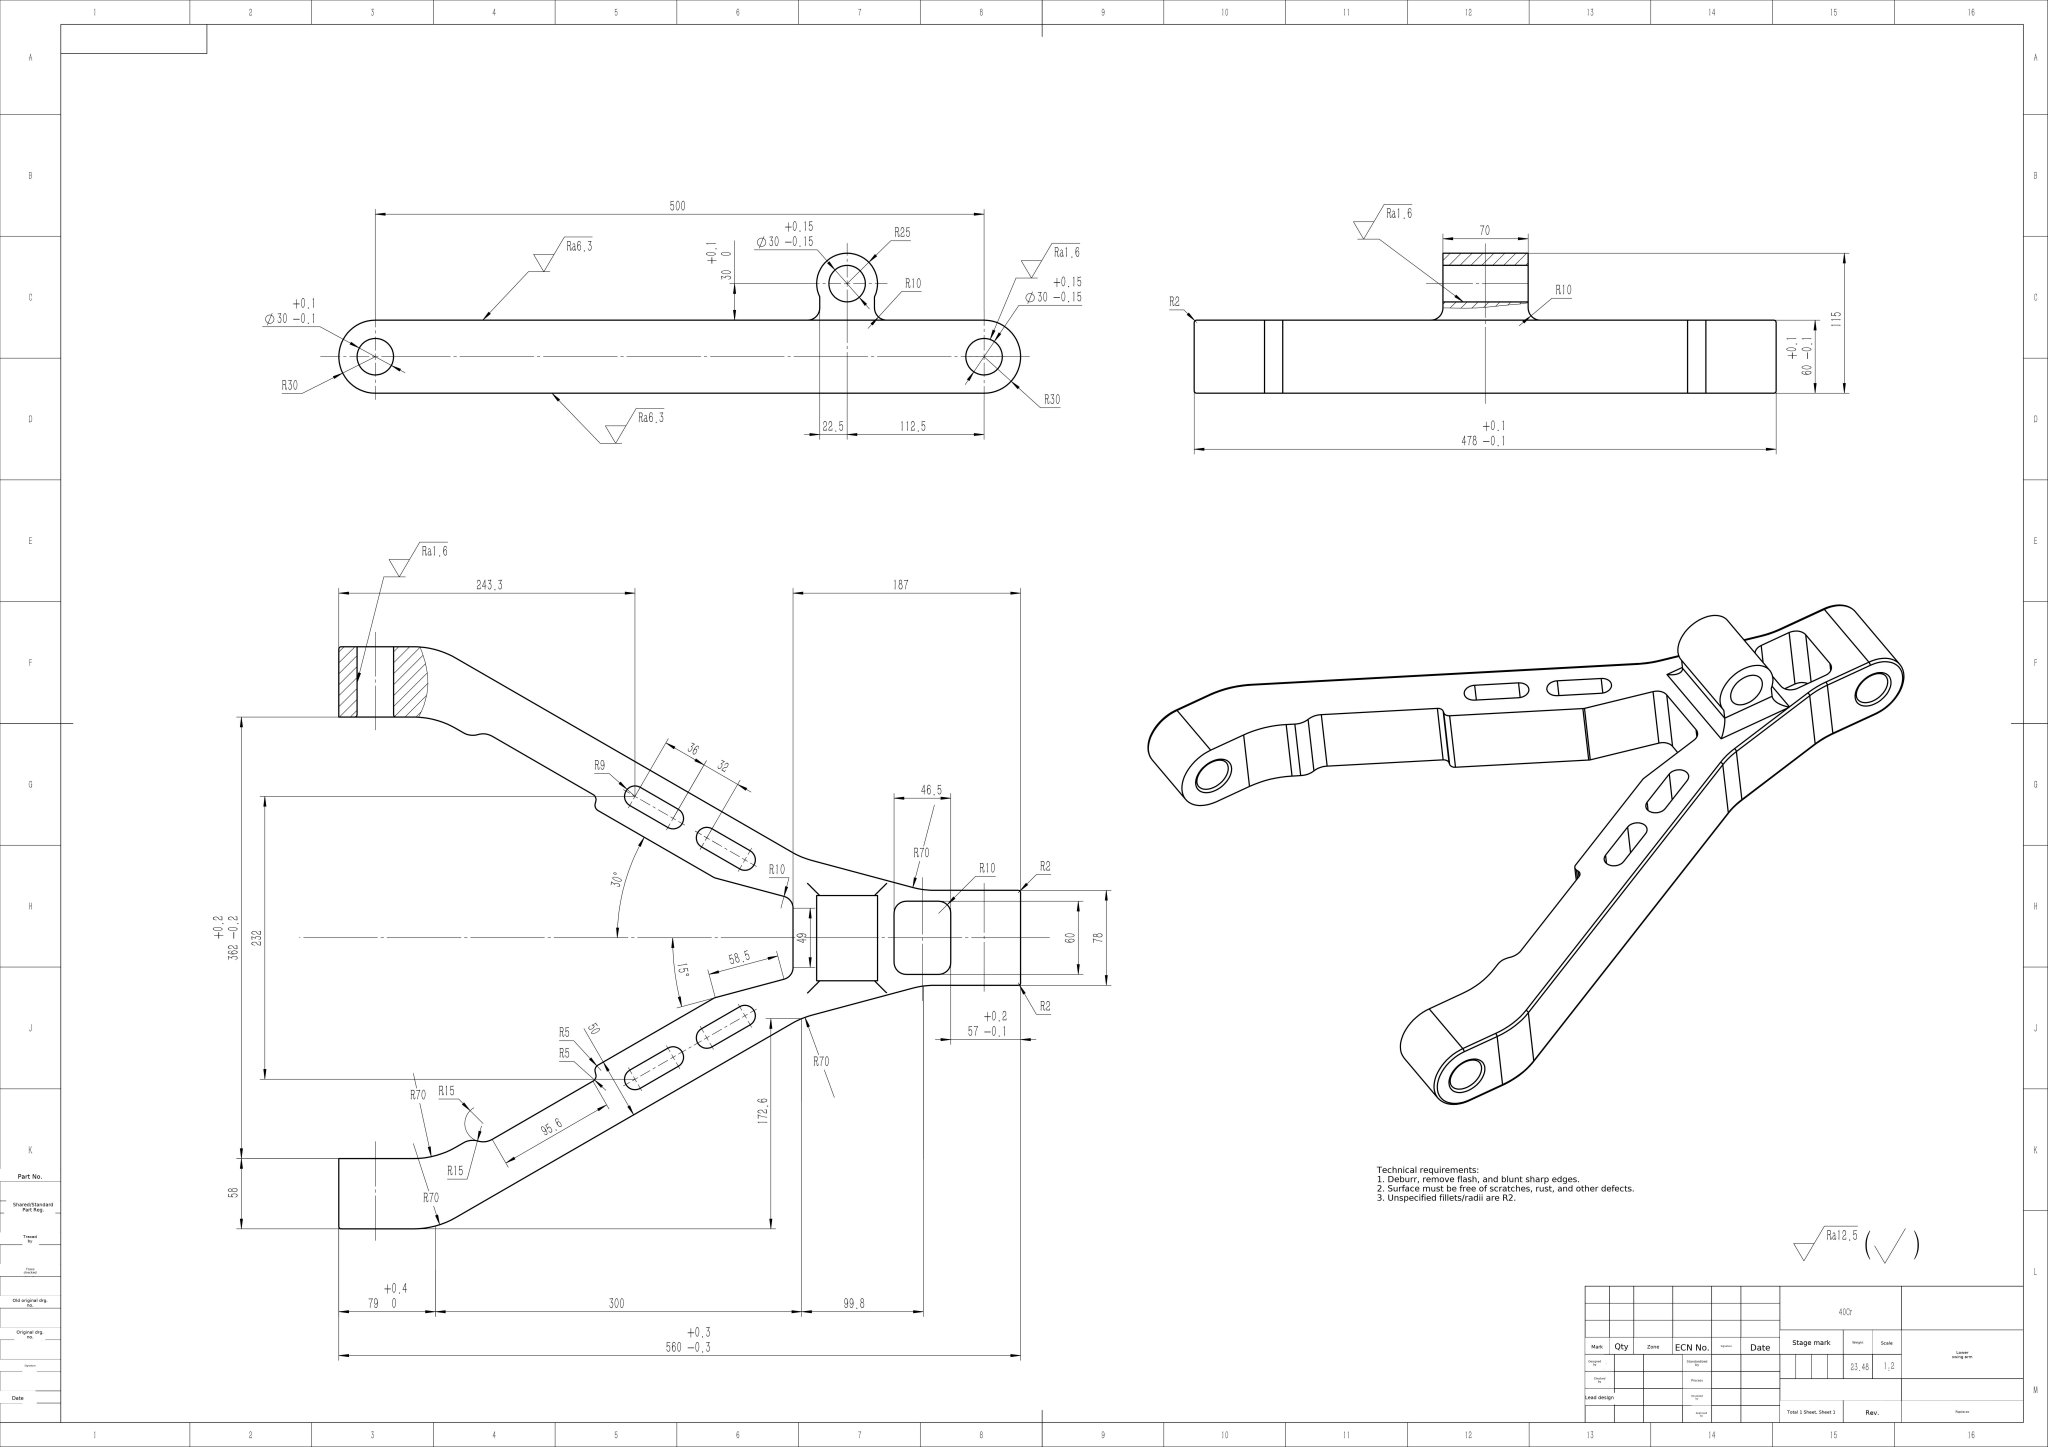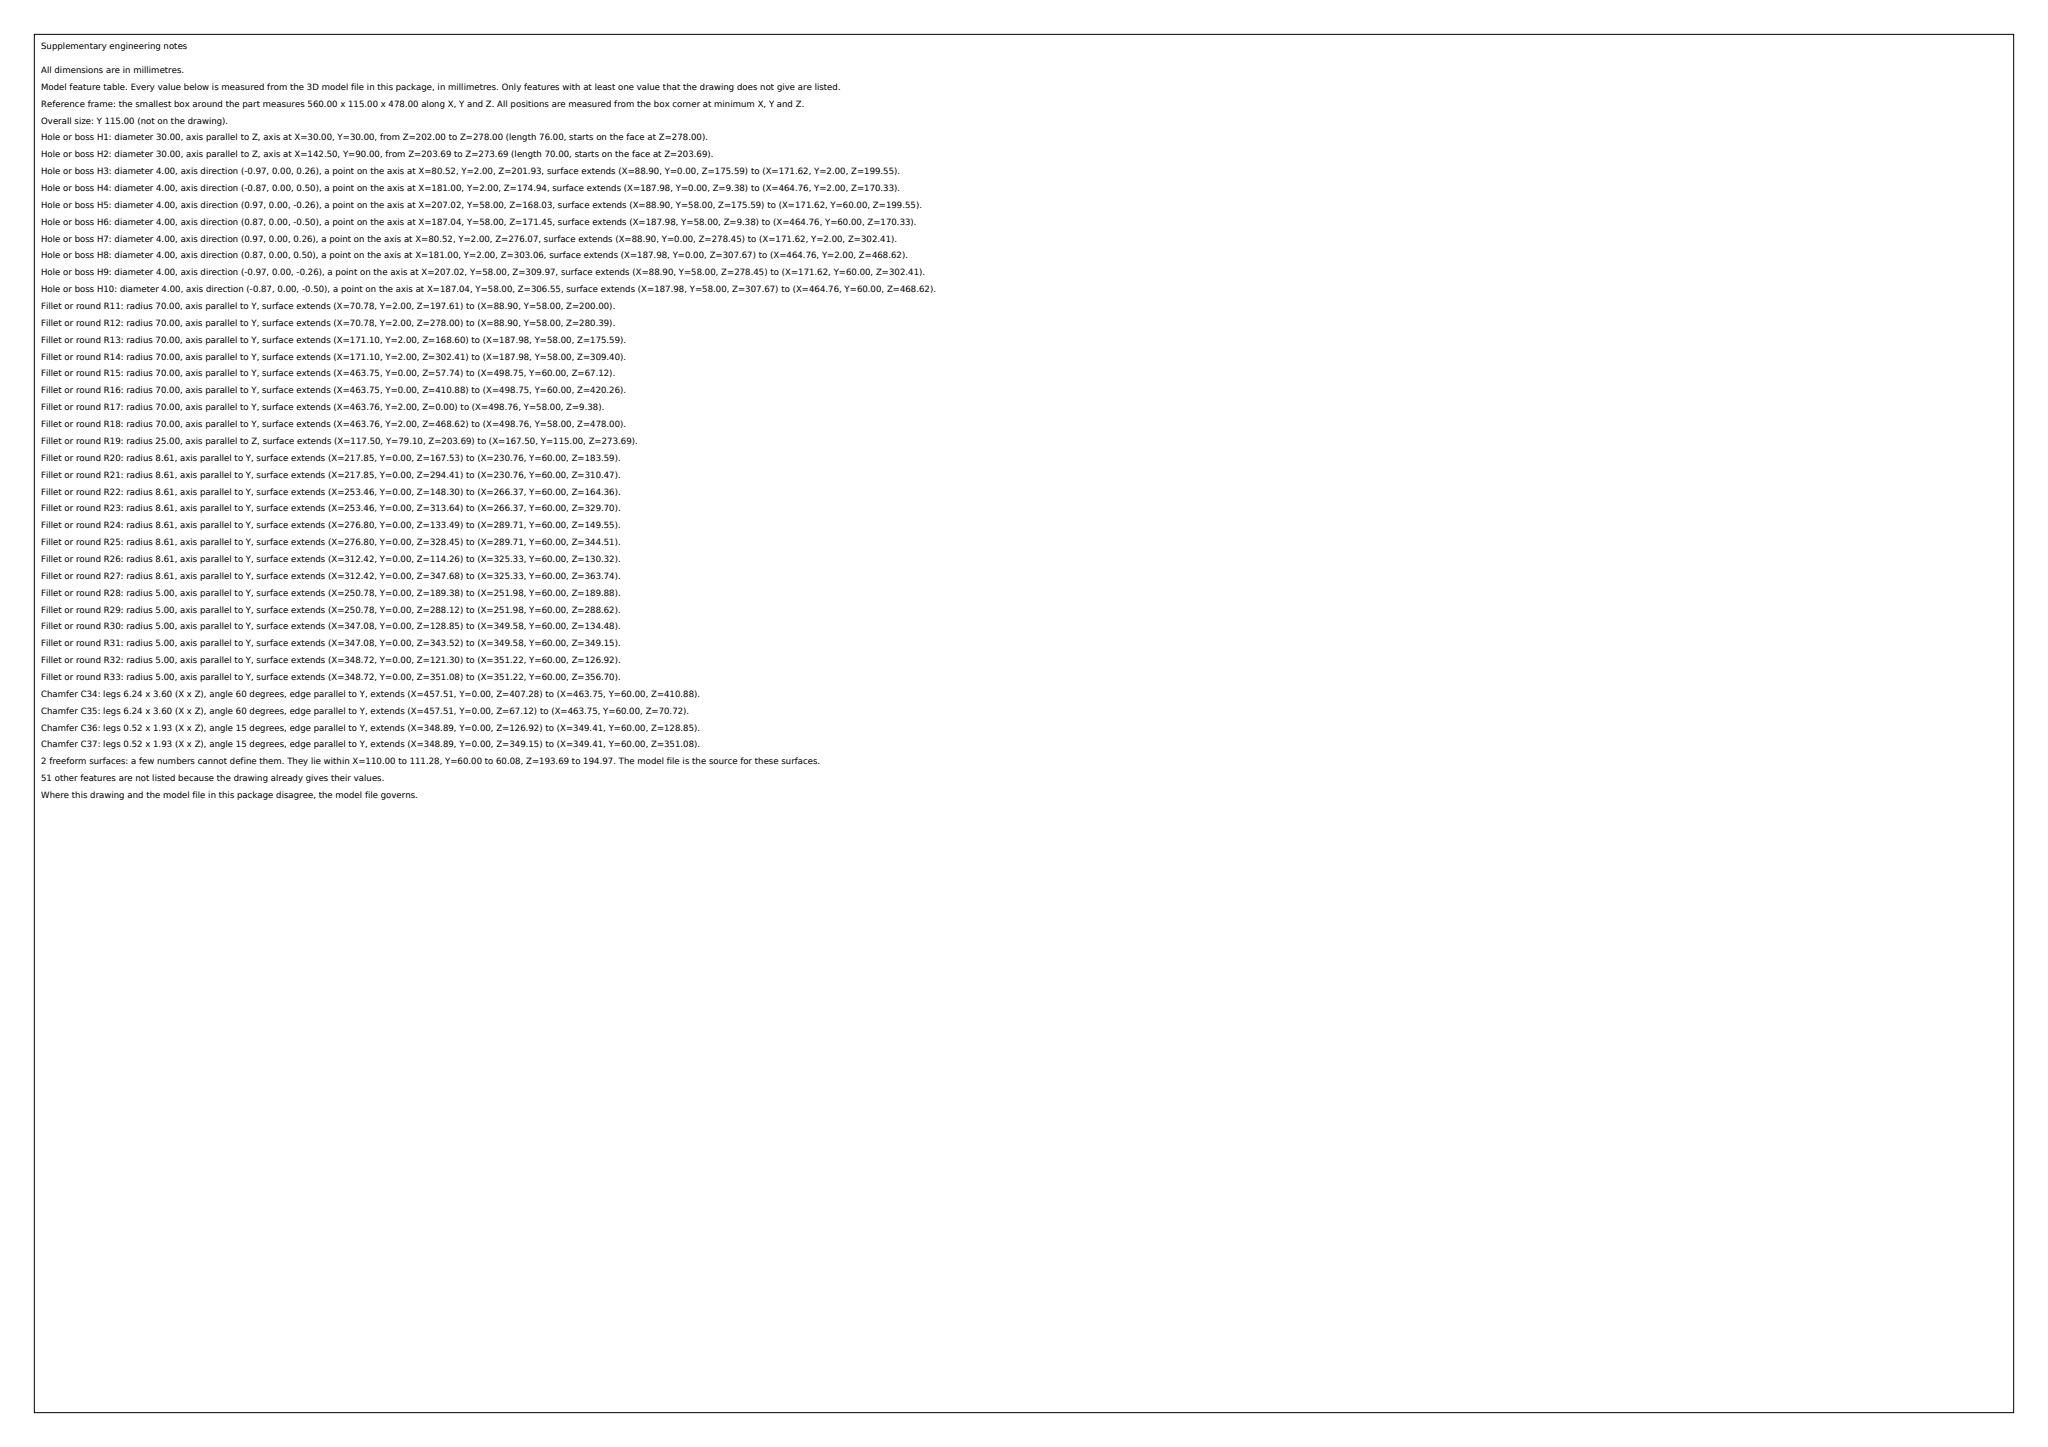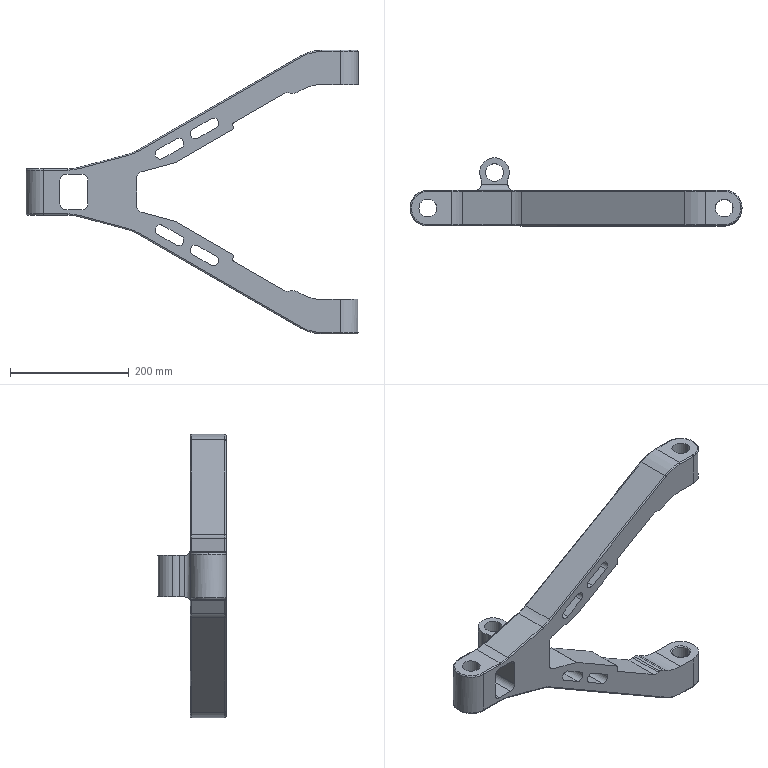Part | SolidWorks | mm | material 400Cr | 1 solid | 140 faces | box 560 x 115 x 478 mm | volume 2983697 mm3 | cylinder 73 | plane 39 | torus 26 | spline 2 | commonest cylinder face diameters 4 x16 30 x14 17.211 x12 20 x10 140 x8 10 x6 60 x4 50 x3